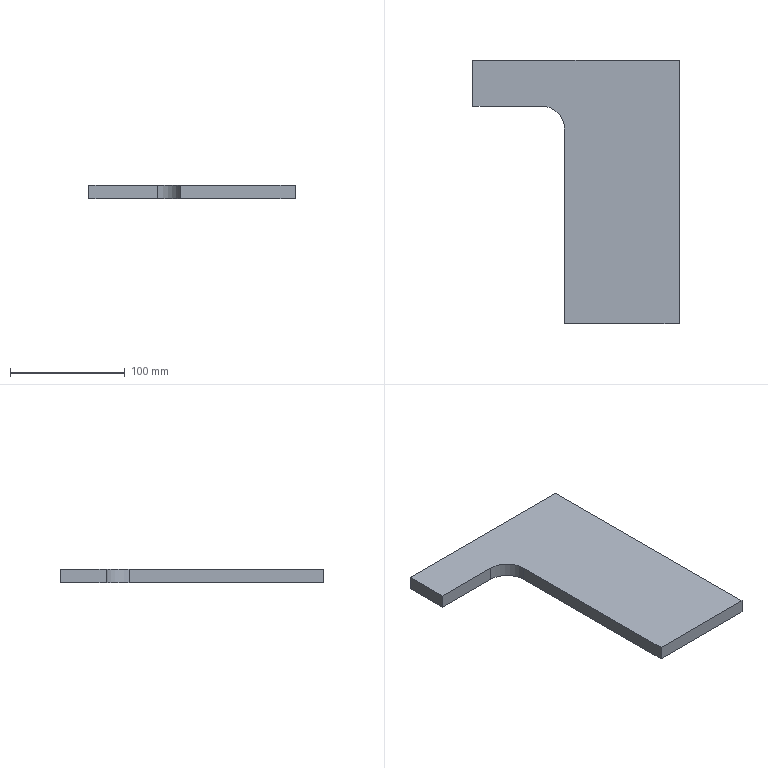Component | SolidWorks | 01-1 | 1 solid | 9 faces | box 180 x 230 x 12 mm | volume 315430 mm3 | plane 8 | cylinder 1 | commonest cylinder face diameters 40 x1
build123d program:
from build123d import *

# Parameters (mm, degrees)
BOSS_EXTRUDE1_DEPTH = 6
FILLET1_R           = 20


with BuildPart() as part:
    # Sketch1 → Boss-Extrude1 (new, symmetric)
    with BuildSketch(Plane.XY):
        Polygon((0, 0), (0, 230), (-180, 230), (-180, 190), (-100, 190), (-100, 0), align=None)
    extrude(amount=BOSS_EXTRUDE1_DEPTH, both=True)

    # Fillet1
    fillet1_edges = [part.edges().sort_by_distance(p)[0] for p in [
        (-100, 190, 0),
    ]]
    fillet(fillet1_edges, radius=FILLET1_R)


solid = part.part
STEP:
#1=CARTESIAN_POINT('',(-3.937,0.,-0.2362));
#2=VERTEX_POINT('',#1);
#3=CARTESIAN_POINT('',(0.,0.,-0.2362));
#4=VERTEX_POINT('',#3);
#5=CARTESIAN_POINT('',(-3.937,0.,-0.2362));
#6=DIRECTION('',(1.,0.,0.));
#7=VECTOR('',#6,39.37);
#8=LINE('',#5,#7);
#9=EDGE_CURVE('',#2,#4,#8,.T.);
#10=ORIENTED_EDGE('',*,*,#9,.T.);
#11=CARTESIAN_POINT('',(0.,0.,0.2362));
#12=VERTEX_POINT('',#11);
#13=CARTESIAN_POINT('',(0.,0.,0.2362));
#14=DIRECTION('',(0.,0.,-1.));
#15=VECTOR('',#14,39.37);
#16=LINE('',#13,#15);
#17=EDGE_CURVE('',#12,#4,#16,.T.);
#18=ORIENTED_EDGE('',*,*,#17,.F.);
#19=CARTESIAN_POINT('',(-3.937,0.,0.2362));
#20=VERTEX_POINT('',#19);
#21=CARTESIAN_POINT('',(-3.937,0.,0.2362));
#22=DIRECTION('',(1.,0.,0.));
#23=VECTOR('',#22,39.37);
#24=LINE('',#21,#23);
#25=EDGE_CURVE('',#20,#12,#24,.T.);
#26=ORIENTED_EDGE('',*,*,#25,.F.);
#27=CARTESIAN_POINT('',(-3.937,0.,0.2362));
#28=DIRECTION('',(0.,0.,-1.));
#29=VECTOR('',#28,39.37);
#30=LINE('',#27,#29);
#31=EDGE_CURVE('',#20,#2,#30,.T.);
#32=ORIENTED_EDGE('',*,*,#31,.T.);
#33=EDGE_LOOP('',(#10,#18,#26,#32));
#34=FACE_OUTER_BOUND('',#33,.T.);
#35=CARTESIAN_POINT('',(-3.937,0.,0.2362));
#36=DIRECTION('',(0.,1.,0.));
#37=DIRECTION('',(0.,0.,1.));
#38=AXIS2_PLACEMENT_3D('',#35,#36,#37);
#39=PLANE('',#38);
#40=ADVANCED_FACE('',(#34),#39,.F.);
#41=CARTESIAN_POINT('',(0.,9.055,-0.2362));
#42=VERTEX_POINT('',#41);
#43=CARTESIAN_POINT('',(0.,0.,-0.2362));
#44=DIRECTION('',(0.,1.,0.));
#45=VECTOR('',#44,39.37);
#46=LINE('',#43,#45);
#47=EDGE_CURVE('',#4,#42,#46,.T.);
#48=ORIENTED_EDGE('',*,*,#47,.T.);
#49=CARTESIAN_POINT('',(0.,9.055,0.2362));
#50=VERTEX_POINT('',#49);
#51=CARTESIAN_POINT('',(0.,9.055,0.2362));
#52=DIRECTION('',(0.,0.,-1.));
#53=VECTOR('',#52,39.37);
#54=LINE('',#51,#53);
#55=EDGE_CURVE('',#50,#42,#54,.T.);
#56=ORIENTED_EDGE('',*,*,#55,.F.);
#57=CARTESIAN_POINT('',(0.,0.,0.2362));
#58=DIRECTION('',(0.,1.,0.));
#59=VECTOR('',#58,39.37);
#60=LINE('',#57,#59);
#61=EDGE_CURVE('',#12,#50,#60,.T.);
#62=ORIENTED_EDGE('',*,*,#61,.F.);
#63=ORIENTED_EDGE('',*,*,#17,.T.);
#64=EDGE_LOOP('',(#48,#56,#62,#63));
#65=FACE_OUTER_BOUND('',#64,.T.);
#66=CARTESIAN_POINT('',(0.,0.,0.2362));
#67=DIRECTION('',(-1.,0.,0.));
#68=DIRECTION('',(0.,0.,1.));
#69=AXIS2_PLACEMENT_3D('',#66,#67,#68);
#70=PLANE('',#69);
#71=ADVANCED_FACE('',(#65),#70,.F.);
#72=CARTESIAN_POINT('',(-7.087,9.055,-0.2362));
#73=VERTEX_POINT('',#72);
#74=CARTESIAN_POINT('',(0.,9.055,-0.2362));
#75=DIRECTION('',(-1.,-0.,0.));
#76=VECTOR('',#75,39.37);
#77=LINE('',#74,#76);
#78=EDGE_CURVE('',#42,#73,#77,.T.);
#79=ORIENTED_EDGE('',*,*,#78,.T.);
#80=CARTESIAN_POINT('',(-7.087,9.055,0.2362));
#81=VERTEX_POINT('',#80);
#82=CARTESIAN_POINT('',(-7.087,9.055,0.2362));
#83=DIRECTION('',(0.,0.,-1.));
#84=VECTOR('',#83,39.37);
#85=LINE('',#82,#84);
#86=EDGE_CURVE('',#81,#73,#85,.T.);
#87=ORIENTED_EDGE('',*,*,#86,.F.);
#88=CARTESIAN_POINT('',(0.,9.055,0.2362));
#89=DIRECTION('',(-1.,-0.,0.));
#90=VECTOR('',#89,39.37);
#91=LINE('',#88,#90);
#92=EDGE_CURVE('',#50,#81,#91,.T.);
#93=ORIENTED_EDGE('',*,*,#92,.F.);
#94=ORIENTED_EDGE('',*,*,#55,.T.);
#95=EDGE_LOOP('',(#79,#87,#93,#94));
#96=FACE_OUTER_BOUND('',#95,.T.);
#97=CARTESIAN_POINT('',(0.,9.055,0.2362));
#98=DIRECTION('',(0.,-1.,0.));
#99=DIRECTION('',(1.,0.,0.));
#100=AXIS2_PLACEMENT_3D('',#97,#98,#99);
#101=PLANE('',#100);
#102=ADVANCED_FACE('',(#96),#101,.F.);
#103=CARTESIAN_POINT('',(-7.087,7.48,-0.2362));
#104=VERTEX_POINT('',#103);
#105=CARTESIAN_POINT('',(-7.087,9.055,-0.2362));
#106=DIRECTION('',(0.,-1.,0.));
#107=VECTOR('',#106,39.37);
#108=LINE('',#105,#107);
#109=EDGE_CURVE('',#73,#104,#108,.T.);
#110=ORIENTED_EDGE('',*,*,#109,.T.);
#111=CARTESIAN_POINT('',(-7.087,7.48,0.2362));
#112=VERTEX_POINT('',#111);
#113=CARTESIAN_POINT('',(-7.087,7.48,0.2362));
#114=DIRECTION('',(0.,0.,-1.));
#115=VECTOR('',#114,39.37);
#116=LINE('',#113,#115);
#117=EDGE_CURVE('',#112,#104,#116,.T.);
#118=ORIENTED_EDGE('',*,*,#117,.F.);
#119=CARTESIAN_POINT('',(-7.087,9.055,0.2362));
#120=DIRECTION('',(0.,-1.,0.));
#121=VECTOR('',#120,39.37);
#122=LINE('',#119,#121);
#123=EDGE_CURVE('',#81,#112,#122,.T.);
#124=ORIENTED_EDGE('',*,*,#123,.F.);
#125=ORIENTED_EDGE('',*,*,#86,.T.);
#126=EDGE_LOOP('',(#110,#118,#124,#125));
#127=FACE_OUTER_BOUND('',#126,.T.);
#128=CARTESIAN_POINT('',(-7.087,9.055,0.2362));
#129=DIRECTION('',(1.,0.,0.));
#130=DIRECTION('',(0.,0.,-1.));
#131=AXIS2_PLACEMENT_3D('',#128,#129,#130);
#132=PLANE('',#131);
#133=ADVANCED_FACE('',(#127),#132,.F.);
#134=CARTESIAN_POINT('',(-4.724,7.48,-0.2362));
#135=VERTEX_POINT('',#134);
#136=CARTESIAN_POINT('',(-7.087,7.48,-0.2362));
#137=DIRECTION('',(1.,0.,0.));
#138=VECTOR('',#137,39.37);
#139=LINE('',#136,#138);
#140=EDGE_CURVE('',#104,#135,#139,.T.);
#141=ORIENTED_EDGE('',*,*,#140,.T.);
#142=CARTESIAN_POINT('',(-4.724,7.48,0.2362));
#143=VERTEX_POINT('',#142);
#144=CARTESIAN_POINT('',(-4.724,7.48,0.2362));
#145=DIRECTION('',(0.,0.,1.));
#146=VECTOR('',#145,39.37);
#147=LINE('',#144,#146);
#148=EDGE_CURVE('',#135,#143,#147,.T.);
#149=ORIENTED_EDGE('',*,*,#148,.T.);
#150=CARTESIAN_POINT('',(-7.087,7.48,0.2362));
#151=DIRECTION('',(1.,0.,0.));
#152=VECTOR('',#151,39.37);
#153=LINE('',#150,#152);
#154=EDGE_CURVE('',#112,#143,#153,.T.);
#155=ORIENTED_EDGE('',*,*,#154,.F.);
#156=ORIENTED_EDGE('',*,*,#117,.T.);
#157=EDGE_LOOP('',(#141,#149,#155,#156));
#158=FACE_OUTER_BOUND('',#157,.T.);
#159=CARTESIAN_POINT('',(-7.087,7.48,0.2362));
#160=DIRECTION('',(0.,1.,0.));
#161=DIRECTION('',(0.,0.,1.));
#162=AXIS2_PLACEMENT_3D('',#159,#160,#161);
#163=PLANE('',#162);
#164=ADVANCED_FACE('',(#158),#163,.F.);
#165=CARTESIAN_POINT('',(-3.937,6.693,0.2362));
#166=VERTEX_POINT('',#165);
#167=CARTESIAN_POINT('',(-3.937,7.48,0.2362));
#168=DIRECTION('',(0.,-1.,0.));
#169=VECTOR('',#168,39.37);
#170=LINE('',#167,#169);
#171=EDGE_CURVE('',#166,#20,#170,.T.);
#172=ORIENTED_EDGE('',*,*,#171,.F.);
#173=CARTESIAN_POINT('',(-3.937,6.693,-0.2362));
#174=VERTEX_POINT('',#173);
#175=CARTESIAN_POINT('',(-3.937,6.693,-0.2362));
#176=DIRECTION('',(0.,0.,-1.));
#177=VECTOR('',#176,39.37);
#178=LINE('',#175,#177);
#179=EDGE_CURVE('',#166,#174,#178,.T.);
#180=ORIENTED_EDGE('',*,*,#179,.T.);
#181=CARTESIAN_POINT('',(-3.937,7.48,-0.2362));
#182=DIRECTION('',(0.,-1.,0.));
#183=VECTOR('',#182,39.37);
#184=LINE('',#181,#183);
#185=EDGE_CURVE('',#174,#2,#184,.T.);
#186=ORIENTED_EDGE('',*,*,#185,.T.);
#187=ORIENTED_EDGE('',*,*,#31,.F.);
#188=EDGE_LOOP('',(#172,#180,#186,#187));
#189=FACE_OUTER_BOUND('',#188,.T.);
#190=CARTESIAN_POINT('',(-3.937,7.48,0.2362));
#191=DIRECTION('',(1.,0.,0.));
#192=DIRECTION('',(-0.,1.,0.));
#193=AXIS2_PLACEMENT_3D('',#190,#191,#192);
#194=PLANE('',#193);
#195=ADVANCED_FACE('',(#189),#194,.F.);
#196=ORIENTED_EDGE('',*,*,#25,.T.);
#197=ORIENTED_EDGE('',*,*,#61,.T.);
#198=ORIENTED_EDGE('',*,*,#92,.T.);
#199=ORIENTED_EDGE('',*,*,#123,.T.);
#200=ORIENTED_EDGE('',*,*,#154,.T.);
#201=CARTESIAN_POINT('',(-4.724,6.693,0.2362));
#202=DIRECTION('',(0.,0.,-1.));
#203=DIRECTION('',(1.,0.,0.));
#204=AXIS2_PLACEMENT_3D('',#201,#202,#203);
#205=CIRCLE('',#204,0.7874);
#206=EDGE_CURVE('',#143,#166,#205,.T.);
#207=ORIENTED_EDGE('',*,*,#206,.T.);
#208=ORIENTED_EDGE('',*,*,#171,.T.);
#209=EDGE_LOOP('',(#196,#197,#198,#199,#200,#207,#208));
#210=FACE_OUTER_BOUND('',#209,.T.);
#211=CARTESIAN_POINT('',(0.,0.,0.2362));
#212=DIRECTION('',(0.,0.,1.));
#213=DIRECTION('',(1.,0.,0.));
#214=AXIS2_PLACEMENT_3D('',#211,#212,#213);
#215=PLANE('',#214);
#216=ADVANCED_FACE('',(#210),#215,.T.);
#217=ORIENTED_EDGE('',*,*,#9,.F.);
#218=ORIENTED_EDGE('',*,*,#185,.F.);
#219=CARTESIAN_POINT('',(-4.724,6.693,-0.2362));
#220=DIRECTION('',(0.,0.,1.));
#221=DIRECTION('',(1.,0.,0.));
#222=AXIS2_PLACEMENT_3D('',#219,#220,#221);
#223=CIRCLE('',#222,0.7874);
#224=EDGE_CURVE('',#174,#135,#223,.T.);
#225=ORIENTED_EDGE('',*,*,#224,.T.);
#226=ORIENTED_EDGE('',*,*,#140,.F.);
#227=ORIENTED_EDGE('',*,*,#109,.F.);
#228=ORIENTED_EDGE('',*,*,#78,.F.);
#229=ORIENTED_EDGE('',*,*,#47,.F.);
#230=EDGE_LOOP('',(#217,#218,#225,#226,#227,#228,#229));
#231=FACE_OUTER_BOUND('',#230,.T.);
#232=CARTESIAN_POINT('',(0.,0.,-0.2362));
#233=DIRECTION('',(0.,0.,1.));
#234=DIRECTION('',(1.,0.,0.));
#235=AXIS2_PLACEMENT_3D('',#232,#233,#234);
#236=PLANE('',#235);
#237=ADVANCED_FACE('',(#231),#236,.F.);
#238=ORIENTED_EDGE('',*,*,#206,.F.);
#239=ORIENTED_EDGE('',*,*,#148,.F.);
#240=ORIENTED_EDGE('',*,*,#224,.F.);
#241=ORIENTED_EDGE('',*,*,#179,.F.);
#242=EDGE_LOOP('',(#238,#239,#240,#241));
#243=FACE_OUTER_BOUND('',#242,.T.);
#244=CARTESIAN_POINT('',(-4.724,6.693,0.2362));
#245=DIRECTION('',(0.,0.,1.));
#246=DIRECTION('',(1.,0.,0.));
#247=AXIS2_PLACEMENT_3D('',#244,#245,#246);
#248=CYLINDRICAL_SURFACE('',#247,0.7874);
#249=ADVANCED_FACE('',(#243),#248,.F.);
#250=CLOSED_SHELL('',(#40,#71,#102,#133,#164,#195,#216,#237,#249));
#251=MANIFOLD_SOLID_BREP('',#250);
#252=CARTESIAN_POINT('',(0.,0.,0.));
#253=DIRECTION('',(0.,0.,1.));
#254=DIRECTION('',(1.,0.,0.));
#255=AXIS2_PLACEMENT_3D('',#252,#253,#254);
#256=(LENGTH_UNIT()NAMED_UNIT(*)SI_UNIT($,.METRE.));
#257=LENGTH_MEASURE_WITH_UNIT(LENGTH_MEASURE(0.0254),#256);
#258=DIMENSIONAL_EXPONENTS(1.,0.,0.,0.,0.,0.,0.);
#259=(CONVERSION_BASED_UNIT('',#257)LENGTH_UNIT()NAMED_UNIT(#258));
#260=UNCERTAINTY_MEASURE_WITH_UNIT(LENGTH_MEASURE(0.00001),#259,'','');
#261=(NAMED_UNIT(*)PLANE_ANGLE_UNIT()SI_UNIT($,.RADIAN.));
#262=(NAMED_UNIT(*)SI_UNIT($,.STERADIAN.)SOLID_ANGLE_UNIT());
#263=(GEOMETRIC_REPRESENTATION_CONTEXT(3)GLOBAL_UNCERTAINTY_ASSIGNED_CONTEXT((#260))GLOBAL_UNIT_ASSIGNED_CONTEXT((#259,#261,#262))REPRESENTATION_CONTEXT('',''));
#264=ADVANCED_BREP_SHAPE_REPRESENTATION('',(#251,#255),#263);
#265=COLOUR_RGB('',0.7922,0.8196,0.9333);
#266=FILL_AREA_STYLE_COLOUR('',#265);
#267=FILL_AREA_STYLE('',(#266));
#268=SURFACE_STYLE_FILL_AREA(#267);
#269=SURFACE_SIDE_STYLE('',(#268));
#270=SURFACE_STYLE_USAGE(.BOTH.,#269);
#271=PRESENTATION_STYLE_ASSIGNMENT((#270));
#272=STYLED_ITEM('',(#271),#251);
#273=PRESENTATION_LAYER_ASSIGNMENT('','',(#272));
#274=(LENGTH_UNIT()NAMED_UNIT(*)SI_UNIT($,.METRE.));
#275=LENGTH_MEASURE_WITH_UNIT(LENGTH_MEASURE(0.0254),#274);
#276=DIMENSIONAL_EXPONENTS(1.,0.,0.,0.,0.,0.,0.);
#277=(CONVERSION_BASED_UNIT('',#275)LENGTH_UNIT()NAMED_UNIT(#276));
#278=UNCERTAINTY_MEASURE_WITH_UNIT(LENGTH_MEASURE(0.00001),#277,'','');
#279=(NAMED_UNIT(*)PLANE_ANGLE_UNIT()SI_UNIT($,.RADIAN.));
#280=(NAMED_UNIT(*)SI_UNIT($,.STERADIAN.)SOLID_ANGLE_UNIT());
#281=(GEOMETRIC_REPRESENTATION_CONTEXT(3)GLOBAL_UNCERTAINTY_ASSIGNED_CONTEXT((#278))GLOBAL_UNIT_ASSIGNED_CONTEXT((#277,#279,#280))REPRESENTATION_CONTEXT('',''));
#282=MECHANICAL_DESIGN_GEOMETRIC_PRESENTATION_REPRESENTATION('',(#272),#281);